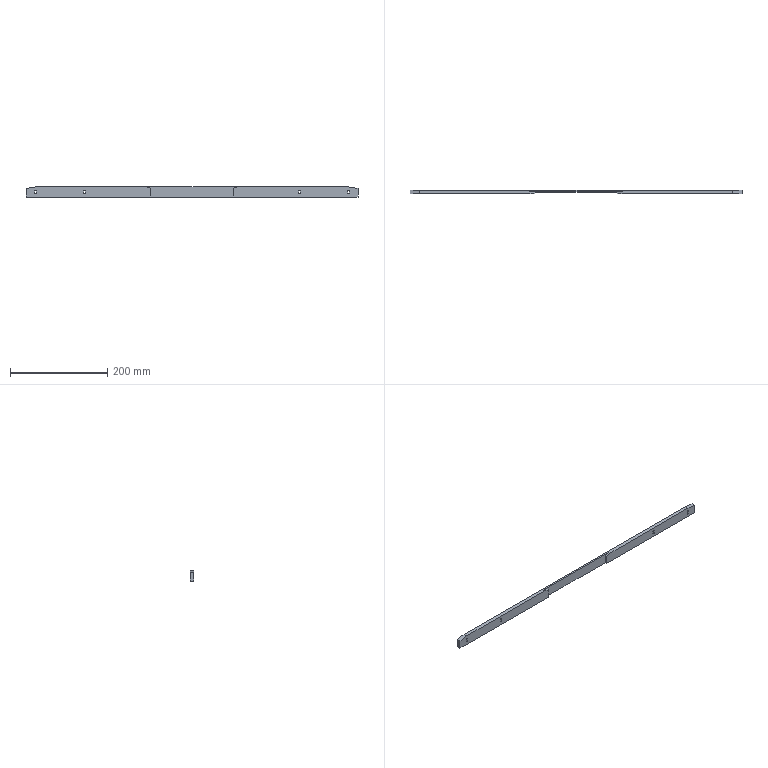Component | SolidWorks | SL010-LeftStreamline-1-1_SL010-02047858StopBarNo.3-1-2 | 1 solid | 30 faces | box 683 x 8 x 21 mm | volume 99149 mm3 | plane 22 | cylinder 8 | commonest cylinder face diameters 3.2 x8 | material White POM
build123d program:
from build123d import *

# Parameters (mm, degrees)
SKETCH1_W           = 683
SKETCH1_H           = 21
BOSS_EXTRUDE1_DEPTH = 8
CUT_EXTRUDE1_DEPTH  = 342.755
CHAMFER1_SIZE       = 3
CHAMFER1_SIZE2      = 20
CHAMFER2_SIZE       = 20
CHAMFER2_SIZE2      = 3
SKETCH4_W           = 169.5
SKETCH4_H           = 4
CUT_EXTRUDE3_DEPTH  = 343.239
CHAMFER3_SIZE       = 10
CHAMFER3_SIZE2      = 2.679


with BuildPart() as part:
    # Sketch1 → Boss-Extrude1 (new body)
    with BuildSketch(Plane.XY):
        Rectangle(SKETCH1_W, SKETCH1_H)
    extrude(amount=BOSS_EXTRUDE1_DEPTH)

    # Sketch2 → Cut-Extrude1 (cut, through all)
    with BuildSketch(Plane.XY.offset(8)):
        with BuildLine():
            Line((223.1, 2.5), (223.1, -2.5))
            ThreePointArc((223.1, -2.5), (221.5, -4.1), (219.9, -2.5))
            Line((219.9, -2.5), (219.9, 2.5))
            ThreePointArc((219.9, 2.5), (221.5, 4.1), (223.1, 2.5))
        make_face()
        with BuildLine():
            Line((323.1, 2.5), (323.1, -2.5))
            ThreePointArc((323.1, -2.5), (321.5, -4.1), (319.9, -2.5))
            Line((319.9, -2.5), (319.9, 2.5))
            ThreePointArc((319.9, 2.5), (321.5, 4.1), (323.1, 2.5))
        make_face()
        with BuildLine():
            Line((-323.1, 2.5), (-323.1, -2.5))
            ThreePointArc((-323.1, -2.5), (-321.5, -4.1), (-319.9, -2.5))
            Line((-319.9, -2.5), (-319.9, 2.5))
            ThreePointArc((-319.9, 2.5), (-321.5, 4.1), (-323.1, 2.5))
        make_face()
        with BuildLine():
            Line((-223.1, 2.5), (-223.1, -2.5))
            ThreePointArc((-223.1, -2.5), (-221.5, -4.1), (-219.9, -2.5))
            Line((-219.9, -2.5), (-219.9, 2.5))
            ThreePointArc((-219.9, 2.5), (-221.5, 4.1), (-223.1, 2.5))
        make_face()
    extrude(amount=-CUT_EXTRUDE1_DEPTH, mode=Mode.SUBTRACT)

    # Chamfer1
    chamfer1_edges = [part.edges().sort_by_distance(p)[0] for p in [
        (341.5, 10.5, 4),
    ]]
    chamfer1_side = [part.faces().sort_by_distance(p)[0] for p in [
        (341.5, 0, 4),
    ]]
    chamfer(chamfer1_edges, length=CHAMFER1_SIZE, length2=CHAMFER1_SIZE2, reference=chamfer1_side[0])

    # Chamfer2
    chamfer2_edges = [part.edges().sort_by_distance(p)[0] for p in [
        (-341.5, 10.5, 4),
    ]]
    chamfer2_side = [part.faces().sort_by_distance(p)[0] for p in [
        (-10, 10.5, 4),
    ]]
    chamfer(chamfer2_edges, length=CHAMFER2_SIZE, length2=CHAMFER2_SIZE2, reference=chamfer2_side[0])

    # Sketch4 → Cut-Extrude3 (cut, through all)
    with BuildSketch(Plane(origin=(0, 10.5, 0), x_dir=(1, 0, 0), z_dir=(0, 1, 0))):
        with Locations((0, -6)):
            Rectangle(SKETCH4_W, SKETCH4_H)
    extrude(amount=-CUT_EXTRUDE3_DEPTH, mode=Mode.SUBTRACT)

    # Chamfer3
    chamfer3_edges = [part.edges().sort_by_distance(p)[0] for p in [
        (-84.75, 10.5, 6),
        (84.75, 10.5, 6),
    ]]
    chamfer3_side = [part.faces().sort_by_distance(p)[0] for p in [
        (0, 10.5, 3.696),
    ]]
    chamfer(chamfer3_edges, length=CHAMFER3_SIZE, length2=CHAMFER3_SIZE2, reference=chamfer3_side[0])


solid = part.part

# Placed as in the assembly
solid = solid.moved(Location((633.5, -101.904, -647.535), (90, 0, 0)))
STEP:
#1=COLOUR_RGB('',0.7922,0.8196,0.9333);
#2=FILL_AREA_STYLE_COLOUR('',#1);
#3=FILL_AREA_STYLE('',(#2));
#4=SURFACE_STYLE_FILL_AREA(#3);
#5=SURFACE_SIDE_STYLE('',(#4));
#6=SURFACE_STYLE_USAGE(.BOTH.,#5);
#7=PRESENTATION_STYLE_ASSIGNMENT((#6));
#8=CARTESIAN_POINT('',(21.604,-4.327,-25.907));
#9=VERTEX_POINT('',#8);
#10=CARTESIAN_POINT('',(21.604,-4.327,-25.186));
#11=VERTEX_POINT('',#10);
#12=CARTESIAN_POINT('',(21.604,-4.327,-25.907));
#13=DIRECTION('',(-0.,-0.,1.));
#14=VECTOR('',#13,39.37);
#15=LINE('',#12,#14);
#16=EDGE_CURVE('',#9,#11,#15,.T.);
#17=ORIENTED_EDGE('',*,*,#16,.T.);
#18=CARTESIAN_POINT('',(21.211,-4.327,-25.08));
#19=VERTEX_POINT('',#18);
#20=CARTESIAN_POINT('',(24.794,-4.327,-26.04));
#21=DIRECTION('',(-0.9659,0.,0.2588));
#22=VECTOR('',#21,39.37);
#23=LINE('',#20,#22);
#24=EDGE_CURVE('',#11,#19,#23,.T.);
#25=ORIENTED_EDGE('',*,*,#24,.T.);
#26=CARTESIAN_POINT('',(12.283,-4.327,-25.08));
#27=VERTEX_POINT('',#26);
#28=CARTESIAN_POINT('',(11.496,-4.327,-25.08));
#29=DIRECTION('',(-1.,0.,-0.));
#30=VECTOR('',#29,39.37);
#31=LINE('',#28,#30);
#32=EDGE_CURVE('',#19,#27,#31,.T.);
#33=ORIENTED_EDGE('',*,*,#32,.T.);
#34=CARTESIAN_POINT('',(11.496,-4.327,-25.198));
#35=VERTEX_POINT('',#34);
#36=CARTESIAN_POINT('',(24.602,-4.327,-23.232));
#37=DIRECTION('',(-0.9889,0.,-0.1483));
#38=VECTOR('',#37,39.37);
#39=LINE('',#36,#38);
#40=EDGE_CURVE('',#27,#35,#39,.T.);
#41=ORIENTED_EDGE('',*,*,#40,.T.);
#42=CARTESIAN_POINT('',(11.496,-4.327,-25.907));
#43=VERTEX_POINT('',#42);
#44=CARTESIAN_POINT('',(11.496,-4.327,-25.08));
#45=DIRECTION('',(0.,0.,-1.));
#46=VECTOR('',#45,39.37);
#47=LINE('',#44,#46);
#48=EDGE_CURVE('',#35,#43,#47,.T.);
#49=ORIENTED_EDGE('',*,*,#48,.T.);
#50=CARTESIAN_POINT('',(11.496,-4.327,-25.907));
#51=DIRECTION('',(1.,-0.,0.));
#52=VECTOR('',#51,39.37);
#53=LINE('',#50,#52);
#54=EDGE_CURVE('',#43,#9,#53,.T.);
#55=ORIENTED_EDGE('',*,*,#54,.T.);
#56=EDGE_LOOP('',(#17,#25,#33,#41,#49,#55));
#57=FACE_OUTER_BOUND('',#56,.T.);
#58=CARTESIAN_POINT('',(12.346,-4.327,-25.395));
#59=VERTEX_POINT('',#58);
#60=CARTESIAN_POINT('',(12.22,-4.327,-25.395));
#61=VERTEX_POINT('',#60);
#62=CARTESIAN_POINT('',(12.283,-4.327,-25.395));
#63=DIRECTION('',(-0.,-1.,0.));
#64=DIRECTION('',(-1.,0.,0.));
#65=AXIS2_PLACEMENT_3D('',#62,#63,#64);
#66=CIRCLE('',#65,0.06299);
#67=EDGE_CURVE('',#59,#61,#66,.T.);
#68=ORIENTED_EDGE('',*,*,#67,.F.);
#69=CARTESIAN_POINT('',(12.346,-4.327,-25.592));
#70=VERTEX_POINT('',#69);
#71=CARTESIAN_POINT('',(12.346,-4.327,-25.395));
#72=DIRECTION('',(-0.,-0.,1.));
#73=VECTOR('',#72,39.37);
#74=LINE('',#71,#73);
#75=EDGE_CURVE('',#70,#59,#74,.T.);
#76=ORIENTED_EDGE('',*,*,#75,.F.);
#77=CARTESIAN_POINT('',(12.22,-4.327,-25.592));
#78=VERTEX_POINT('',#77);
#79=CARTESIAN_POINT('',(12.283,-4.327,-25.592));
#80=DIRECTION('',(-0.,-1.,0.));
#81=DIRECTION('',(-1.,0.,0.));
#82=AXIS2_PLACEMENT_3D('',#79,#80,#81);
#83=CIRCLE('',#82,0.06299);
#84=EDGE_CURVE('',#78,#70,#83,.T.);
#85=ORIENTED_EDGE('',*,*,#84,.F.);
#86=CARTESIAN_POINT('',(12.22,-4.327,-25.395));
#87=DIRECTION('',(0.,0.,-1.));
#88=VECTOR('',#87,39.37);
#89=LINE('',#86,#88);
#90=EDGE_CURVE('',#61,#78,#89,.T.);
#91=ORIENTED_EDGE('',*,*,#90,.F.);
#92=EDGE_LOOP('',(#68,#76,#85,#91));
#93=FACE_BOUND('',#92,.T.);
#94=CARTESIAN_POINT('',(16.283,-4.327,-25.395));
#95=VERTEX_POINT('',#94);
#96=CARTESIAN_POINT('',(16.157,-4.327,-25.395));
#97=VERTEX_POINT('',#96);
#98=CARTESIAN_POINT('',(16.22,-4.327,-25.395));
#99=DIRECTION('',(-0.,-1.,0.));
#100=DIRECTION('',(-1.,0.,0.));
#101=AXIS2_PLACEMENT_3D('',#98,#99,#100);
#102=CIRCLE('',#101,0.06299);
#103=EDGE_CURVE('',#95,#97,#102,.T.);
#104=ORIENTED_EDGE('',*,*,#103,.F.);
#105=CARTESIAN_POINT('',(16.283,-4.327,-25.592));
#106=VERTEX_POINT('',#105);
#107=CARTESIAN_POINT('',(16.283,-4.327,-25.395));
#108=DIRECTION('',(-0.,-0.,1.));
#109=VECTOR('',#108,39.37);
#110=LINE('',#107,#109);
#111=EDGE_CURVE('',#106,#95,#110,.T.);
#112=ORIENTED_EDGE('',*,*,#111,.F.);
#113=CARTESIAN_POINT('',(16.157,-4.327,-25.592));
#114=VERTEX_POINT('',#113);
#115=CARTESIAN_POINT('',(16.22,-4.327,-25.592));
#116=DIRECTION('',(-0.,-1.,0.));
#117=DIRECTION('',(-1.,0.,0.));
#118=AXIS2_PLACEMENT_3D('',#115,#116,#117);
#119=CIRCLE('',#118,0.06299);
#120=EDGE_CURVE('',#114,#106,#119,.T.);
#121=ORIENTED_EDGE('',*,*,#120,.F.);
#122=CARTESIAN_POINT('',(16.157,-4.327,-25.395));
#123=DIRECTION('',(0.,0.,-1.));
#124=VECTOR('',#123,39.37);
#125=LINE('',#122,#124);
#126=EDGE_CURVE('',#97,#114,#125,.T.);
#127=ORIENTED_EDGE('',*,*,#126,.F.);
#128=EDGE_LOOP('',(#104,#112,#121,#127));
#129=FACE_BOUND('',#128,.T.);
#130=CARTESIAN_POINT('',(24.941,-4.327,-25.494));
#131=DIRECTION('',(-0.,-1.,0.));
#132=DIRECTION('',(1.,-0.,0.));
#133=AXIS2_PLACEMENT_3D('',#130,#131,#132);
#134=PLANE('',#133);
#135=ADVANCED_FACE('',(#57,#93,#129),#134,.T.);
#136=CARTESIAN_POINT('',(38.386,-4.012,-25.907));
#137=VERTEX_POINT('',#136);
#138=CARTESIAN_POINT('',(38.386,-4.012,-25.198));
#139=VERTEX_POINT('',#138);
#140=CARTESIAN_POINT('',(38.386,-4.012,-25.08));
#141=DIRECTION('',(-0.,-0.,1.));
#142=VECTOR('',#141,39.37);
#143=LINE('',#140,#142);
#144=EDGE_CURVE('',#137,#139,#143,.T.);
#145=ORIENTED_EDGE('',*,*,#144,.T.);
#146=CARTESIAN_POINT('',(38.386,-4.327,-25.198));
#147=VERTEX_POINT('',#146);
#148=CARTESIAN_POINT('',(38.386,-4.327,-25.198));
#149=DIRECTION('',(-0.,-1.,0.));
#150=VECTOR('',#149,39.37);
#151=LINE('',#148,#150);
#152=EDGE_CURVE('',#139,#147,#151,.T.);
#153=ORIENTED_EDGE('',*,*,#152,.T.);
#154=CARTESIAN_POINT('',(38.386,-4.327,-25.907));
#155=VERTEX_POINT('',#154);
#156=CARTESIAN_POINT('',(38.386,-4.327,-25.08));
#157=DIRECTION('',(-0.,-0.,1.));
#158=VECTOR('',#157,39.37);
#159=LINE('',#156,#158);
#160=EDGE_CURVE('',#155,#147,#159,.T.);
#161=ORIENTED_EDGE('',*,*,#160,.F.);
#162=CARTESIAN_POINT('',(38.386,-4.327,-25.907));
#163=DIRECTION('',(0.,1.,-0.));
#164=VECTOR('',#163,39.37);
#165=LINE('',#162,#164);
#166=EDGE_CURVE('',#155,#137,#165,.T.);
#167=ORIENTED_EDGE('',*,*,#166,.T.);
#168=EDGE_LOOP('',(#145,#153,#161,#167));
#169=FACE_OUTER_BOUND('',#168,.T.);
#170=CARTESIAN_POINT('',(38.386,-4.327,-25.08));
#171=DIRECTION('',(-1.,0.,-0.));
#172=DIRECTION('',(-0.,-1.,0.));
#173=AXIS2_PLACEMENT_3D('',#170,#171,#172);
#174=PLANE('',#173);
#175=ADVANCED_FACE('',(#169),#174,.F.);
#176=CARTESIAN_POINT('',(28.671,-4.169,-25.08));
#177=VERTEX_POINT('',#176);
#178=CARTESIAN_POINT('',(21.211,-4.169,-25.08));
#179=VERTEX_POINT('',#178);
#180=CARTESIAN_POINT('',(21.604,-4.169,-25.08));
#181=DIRECTION('',(-1.,-0.,-0.));
#182=VECTOR('',#181,39.37);
#183=LINE('',#180,#182);
#184=EDGE_CURVE('',#177,#179,#183,.T.);
#185=ORIENTED_EDGE('',*,*,#184,.F.);
#186=CARTESIAN_POINT('',(28.671,-4.327,-25.08));
#187=VERTEX_POINT('',#186);
#188=CARTESIAN_POINT('',(28.671,-4.327,-25.08));
#189=DIRECTION('',(-0.,-1.,0.));
#190=VECTOR('',#189,39.37);
#191=LINE('',#188,#190);
#192=EDGE_CURVE('',#177,#187,#191,.T.);
#193=ORIENTED_EDGE('',*,*,#192,.T.);
#194=CARTESIAN_POINT('',(37.598,-4.327,-25.08));
#195=VERTEX_POINT('',#194);
#196=CARTESIAN_POINT('',(11.496,-4.327,-25.08));
#197=DIRECTION('',(-1.,0.,-0.));
#198=VECTOR('',#197,39.37);
#199=LINE('',#196,#198);
#200=EDGE_CURVE('',#195,#187,#199,.T.);
#201=ORIENTED_EDGE('',*,*,#200,.F.);
#202=CARTESIAN_POINT('',(37.598,-4.012,-25.08));
#203=VERTEX_POINT('',#202);
#204=CARTESIAN_POINT('',(37.598,-4.327,-25.08));
#205=DIRECTION('',(0.,1.,-0.));
#206=VECTOR('',#205,39.37);
#207=LINE('',#204,#206);
#208=EDGE_CURVE('',#195,#203,#207,.T.);
#209=ORIENTED_EDGE('',*,*,#208,.T.);
#210=CARTESIAN_POINT('',(12.283,-4.012,-25.08));
#211=VERTEX_POINT('',#210);
#212=CARTESIAN_POINT('',(11.496,-4.012,-25.08));
#213=DIRECTION('',(-1.,0.,-0.));
#214=VECTOR('',#213,39.37);
#215=LINE('',#212,#214);
#216=EDGE_CURVE('',#203,#211,#215,.T.);
#217=ORIENTED_EDGE('',*,*,#216,.T.);
#218=CARTESIAN_POINT('',(12.283,-4.327,-25.08));
#219=DIRECTION('',(-0.,-1.,0.));
#220=VECTOR('',#219,39.37);
#221=LINE('',#218,#220);
#222=EDGE_CURVE('',#211,#27,#221,.T.);
#223=ORIENTED_EDGE('',*,*,#222,.T.);
#224=ORIENTED_EDGE('',*,*,#32,.F.);
#225=CARTESIAN_POINT('',(21.211,-4.327,-25.08));
#226=DIRECTION('',(0.,1.,-0.));
#227=VECTOR('',#226,39.37);
#228=LINE('',#225,#227);
#229=EDGE_CURVE('',#19,#179,#228,.T.);
#230=ORIENTED_EDGE('',*,*,#229,.T.);
#231=EDGE_LOOP('',(#185,#193,#201,#209,#217,#223,#224,#230));
#232=FACE_OUTER_BOUND('',#231,.T.);
#233=CARTESIAN_POINT('',(11.496,-4.327,-25.08));
#234=DIRECTION('',(0.,-0.,-1.));
#235=DIRECTION('',(0.,1.,-0.));
#236=AXIS2_PLACEMENT_3D('',#233,#234,#235);
#237=PLANE('',#236);
#238=ADVANCED_FACE('',(#232),#237,.F.);
#239=ORIENTED_EDGE('',*,*,#48,.F.);
#240=CARTESIAN_POINT('',(11.496,-4.012,-25.198));
#241=VERTEX_POINT('',#240);
#242=CARTESIAN_POINT('',(11.496,-4.327,-25.198));
#243=DIRECTION('',(0.,1.,-0.));
#244=VECTOR('',#243,39.37);
#245=LINE('',#242,#244);
#246=EDGE_CURVE('',#35,#241,#245,.T.);
#247=ORIENTED_EDGE('',*,*,#246,.T.);
#248=CARTESIAN_POINT('',(11.496,-4.012,-25.907));
#249=VERTEX_POINT('',#248);
#250=CARTESIAN_POINT('',(11.496,-4.012,-25.08));
#251=DIRECTION('',(0.,0.,-1.));
#252=VECTOR('',#251,39.37);
#253=LINE('',#250,#252);
#254=EDGE_CURVE('',#241,#249,#253,.T.);
#255=ORIENTED_EDGE('',*,*,#254,.T.);
#256=CARTESIAN_POINT('',(11.496,-4.327,-25.907));
#257=DIRECTION('',(0.,1.,-0.));
#258=VECTOR('',#257,39.37);
#259=LINE('',#256,#258);
#260=EDGE_CURVE('',#43,#249,#259,.T.);
#261=ORIENTED_EDGE('',*,*,#260,.F.);
#262=EDGE_LOOP('',(#239,#247,#255,#261));
#263=FACE_OUTER_BOUND('',#262,.T.);
#264=CARTESIAN_POINT('',(11.496,-4.327,-25.08));
#265=DIRECTION('',(1.,-0.,0.));
#266=DIRECTION('',(0.,1.,-0.));
#267=AXIS2_PLACEMENT_3D('',#264,#265,#266);
#268=PLANE('',#267);
#269=ADVANCED_FACE('',(#263),#268,.F.);
#270=CARTESIAN_POINT('',(28.278,-4.169,-25.907));
#271=VERTEX_POINT('',#270);
#272=CARTESIAN_POINT('',(21.604,-4.169,-25.907));
#273=VERTEX_POINT('',#272);
#274=CARTESIAN_POINT('',(21.604,-4.169,-25.907));
#275=DIRECTION('',(-1.,-0.,-0.));
#276=VECTOR('',#275,39.37);
#277=LINE('',#274,#276);
#278=EDGE_CURVE('',#271,#273,#277,.T.);
#279=ORIENTED_EDGE('',*,*,#278,.T.);
#280=CARTESIAN_POINT('',(21.604,-4.327,-25.907));
#281=DIRECTION('',(-0.,-1.,0.));
#282=VECTOR('',#281,39.37);
#283=LINE('',#280,#282);
#284=EDGE_CURVE('',#273,#9,#283,.T.);
#285=ORIENTED_EDGE('',*,*,#284,.T.);
#286=ORIENTED_EDGE('',*,*,#54,.F.);
#287=ORIENTED_EDGE('',*,*,#260,.T.);
#288=CARTESIAN_POINT('',(11.496,-4.012,-25.907));
#289=DIRECTION('',(1.,-0.,0.));
#290=VECTOR('',#289,39.37);
#291=LINE('',#288,#290);
#292=EDGE_CURVE('',#249,#137,#291,.T.);
#293=ORIENTED_EDGE('',*,*,#292,.T.);
#294=ORIENTED_EDGE('',*,*,#166,.F.);
#295=CARTESIAN_POINT('',(28.278,-4.327,-25.907));
#296=VERTEX_POINT('',#295);
#297=CARTESIAN_POINT('',(11.496,-4.327,-25.907));
#298=DIRECTION('',(1.,-0.,0.));
#299=VECTOR('',#298,39.37);
#300=LINE('',#297,#299);
#301=EDGE_CURVE('',#296,#155,#300,.T.);
#302=ORIENTED_EDGE('',*,*,#301,.F.);
#303=CARTESIAN_POINT('',(28.278,-4.327,-25.907));
#304=DIRECTION('',(0.,1.,-0.));
#305=VECTOR('',#304,39.37);
#306=LINE('',#303,#305);
#307=EDGE_CURVE('',#296,#271,#306,.T.);
#308=ORIENTED_EDGE('',*,*,#307,.T.);
#309=EDGE_LOOP('',(#279,#285,#286,#287,#293,#294,#302,#308));
#310=FACE_OUTER_BOUND('',#309,.T.);
#311=CARTESIAN_POINT('',(11.496,-4.327,-25.907));
#312=DIRECTION('',(-0.,0.,1.));
#313=DIRECTION('',(-0.,-1.,0.));
#314=AXIS2_PLACEMENT_3D('',#311,#312,#313);
#315=PLANE('',#314);
#316=ADVANCED_FACE('',(#310),#315,.F.);
#317=ORIENTED_EDGE('',*,*,#200,.T.);
#318=CARTESIAN_POINT('',(28.278,-4.327,-25.186));
#319=VERTEX_POINT('',#318);
#320=CARTESIAN_POINT('',(25.087,-4.327,-26.04));
#321=DIRECTION('',(-0.9659,0.,-0.2588));
#322=VECTOR('',#321,39.37);
#323=LINE('',#320,#322);
#324=EDGE_CURVE('',#187,#319,#323,.T.);
#325=ORIENTED_EDGE('',*,*,#324,.T.);
#326=CARTESIAN_POINT('',(28.278,-4.327,-25.907));
#327=DIRECTION('',(-0.,-0.,1.));
#328=VECTOR('',#327,39.37);
#329=LINE('',#326,#328);
#330=EDGE_CURVE('',#296,#319,#329,.T.);
#331=ORIENTED_EDGE('',*,*,#330,.F.);
#332=ORIENTED_EDGE('',*,*,#301,.T.);
#333=ORIENTED_EDGE('',*,*,#160,.T.);
#334=CARTESIAN_POINT('',(25.28,-4.327,-23.232));
#335=DIRECTION('',(-0.9889,0.,0.1483));
#336=VECTOR('',#335,39.37);
#337=LINE('',#334,#336);
#338=EDGE_CURVE('',#147,#195,#337,.T.);
#339=ORIENTED_EDGE('',*,*,#338,.T.);
#340=EDGE_LOOP('',(#317,#325,#331,#332,#333,#339));
#341=FACE_OUTER_BOUND('',#340,.T.);
#342=CARTESIAN_POINT('',(37.661,-4.327,-25.395));
#343=VERTEX_POINT('',#342);
#344=CARTESIAN_POINT('',(37.535,-4.327,-25.395));
#345=VERTEX_POINT('',#344);
#346=CARTESIAN_POINT('',(37.598,-4.327,-25.395));
#347=DIRECTION('',(-0.,-1.,0.));
#348=DIRECTION('',(1.,0.,0.));
#349=AXIS2_PLACEMENT_3D('',#346,#347,#348);
#350=CIRCLE('',#349,0.06299);
#351=EDGE_CURVE('',#343,#345,#350,.T.);
#352=ORIENTED_EDGE('',*,*,#351,.F.);
#353=CARTESIAN_POINT('',(37.661,-4.327,-25.592));
#354=VERTEX_POINT('',#353);
#355=CARTESIAN_POINT('',(37.661,-4.327,-25.395));
#356=DIRECTION('',(-0.,-0.,1.));
#357=VECTOR('',#356,39.37);
#358=LINE('',#355,#357);
#359=EDGE_CURVE('',#354,#343,#358,.T.);
#360=ORIENTED_EDGE('',*,*,#359,.F.);
#361=CARTESIAN_POINT('',(37.535,-4.327,-25.592));
#362=VERTEX_POINT('',#361);
#363=CARTESIAN_POINT('',(37.598,-4.327,-25.592));
#364=DIRECTION('',(-0.,-1.,0.));
#365=DIRECTION('',(1.,0.,0.));
#366=AXIS2_PLACEMENT_3D('',#363,#364,#365);
#367=CIRCLE('',#366,0.06299);
#368=EDGE_CURVE('',#362,#354,#367,.T.);
#369=ORIENTED_EDGE('',*,*,#368,.F.);
#370=CARTESIAN_POINT('',(37.535,-4.327,-25.395));
#371=DIRECTION('',(0.,0.,-1.));
#372=VECTOR('',#371,39.37);
#373=LINE('',#370,#372);
#374=EDGE_CURVE('',#345,#362,#373,.T.);
#375=ORIENTED_EDGE('',*,*,#374,.F.);
#376=EDGE_LOOP('',(#352,#360,#369,#375));
#377=FACE_BOUND('',#376,.T.);
#378=CARTESIAN_POINT('',(33.724,-4.327,-25.395));
#379=VERTEX_POINT('',#378);
#380=CARTESIAN_POINT('',(33.598,-4.327,-25.395));
#381=VERTEX_POINT('',#380);
#382=CARTESIAN_POINT('',(33.661,-4.327,-25.395));
#383=DIRECTION('',(-0.,-1.,0.));
#384=DIRECTION('',(1.,0.,0.));
#385=AXIS2_PLACEMENT_3D('',#382,#383,#384);
#386=CIRCLE('',#385,0.06299);
#387=EDGE_CURVE('',#379,#381,#386,.T.);
#388=ORIENTED_EDGE('',*,*,#387,.F.);
#389=CARTESIAN_POINT('',(33.724,-4.327,-25.592));
#390=VERTEX_POINT('',#389);
#391=CARTESIAN_POINT('',(33.724,-4.327,-25.395));
#392=DIRECTION('',(-0.,-0.,1.));
#393=VECTOR('',#392,39.37);
#394=LINE('',#391,#393);
#395=EDGE_CURVE('',#390,#379,#394,.T.);
#396=ORIENTED_EDGE('',*,*,#395,.F.);
#397=CARTESIAN_POINT('',(33.598,-4.327,-25.592));
#398=VERTEX_POINT('',#397);
#399=CARTESIAN_POINT('',(33.661,-4.327,-25.592));
#400=DIRECTION('',(-0.,-1.,0.));
#401=DIRECTION('',(1.,0.,0.));
#402=AXIS2_PLACEMENT_3D('',#399,#400,#401);
#403=CIRCLE('',#402,0.06299);
#404=EDGE_CURVE('',#398,#390,#403,.T.);
#405=ORIENTED_EDGE('',*,*,#404,.F.);
#406=CARTESIAN_POINT('',(33.598,-4.327,-25.395));
#407=DIRECTION('',(0.,0.,-1.));
#408=VECTOR('',#407,39.37);
#409=LINE('',#406,#408);
#410=EDGE_CURVE('',#381,#398,#409,.T.);
#411=ORIENTED_EDGE('',*,*,#410,.F.);
#412=EDGE_LOOP('',(#388,#396,#405,#411));
#413=FACE_BOUND('',#412,.T.);
#414=CARTESIAN_POINT('',(24.941,-4.327,-25.494));
#415=DIRECTION('',(-0.,-1.,0.));
#416=DIRECTION('',(1.,-0.,0.));
#417=AXIS2_PLACEMENT_3D('',#414,#415,#416);
#418=PLANE('',#417);
#419=ADVANCED_FACE('',(#341,#377,#413),#418,.T.);
#420=CARTESIAN_POINT('',(16.283,-4.012,-25.592));
#421=VERTEX_POINT('',#420);
#422=CARTESIAN_POINT('',(16.283,-4.012,-25.395));
#423=VERTEX_POINT('',#422);
#424=CARTESIAN_POINT('',(16.283,-4.012,-25.395));
#425=DIRECTION('',(-0.,-0.,1.));
#426=VECTOR('',#425,39.37);
#427=LINE('',#424,#426);
#428=EDGE_CURVE('',#421,#423,#427,.T.);
#429=ORIENTED_EDGE('',*,*,#428,.T.);
#430=CARTESIAN_POINT('',(16.157,-4.012,-25.395));
#431=VERTEX_POINT('',#430);
#432=CARTESIAN_POINT('',(16.22,-4.012,-25.395));
#433=DIRECTION('',(-0.,-1.,0.));
#434=DIRECTION('',(-1.,0.,0.));
#435=AXIS2_PLACEMENT_3D('',#432,#433,#434);
#436=CIRCLE('',#435,0.06299);
#437=EDGE_CURVE('',#423,#431,#436,.T.);
#438=ORIENTED_EDGE('',*,*,#437,.T.);
#439=CARTESIAN_POINT('',(16.157,-4.012,-25.592));
#440=VERTEX_POINT('',#439);
#441=CARTESIAN_POINT('',(16.157,-4.012,-25.395));
#442=DIRECTION('',(0.,0.,-1.));
#443=VECTOR('',#442,39.37);
#444=LINE('',#441,#443);
#445=EDGE_CURVE('',#431,#440,#444,.T.);
#446=ORIENTED_EDGE('',*,*,#445,.T.);
#447=CARTESIAN_POINT('',(16.22,-4.012,-25.592));
#448=DIRECTION('',(-0.,-1.,0.));
#449=DIRECTION('',(-1.,0.,0.));
#450=AXIS2_PLACEMENT_3D('',#447,#448,#449);
#451=CIRCLE('',#450,0.06299);
#452=EDGE_CURVE('',#440,#421,#451,.T.);
#453=ORIENTED_EDGE('',*,*,#452,.T.);
#454=EDGE_LOOP('',(#429,#438,#446,#453));
#455=FACE_BOUND('',#454,.T.);
#456=CARTESIAN_POINT('',(12.346,-4.012,-25.592));
#457=VERTEX_POINT('',#456);
#458=CARTESIAN_POINT('',(12.346,-4.012,-25.395));
#459=VERTEX_POINT('',#458);
#460=CARTESIAN_POINT('',(12.346,-4.012,-25.395));
#461=DIRECTION('',(-0.,-0.,1.));
#462=VECTOR('',#461,39.37);
#463=LINE('',#460,#462);
#464=EDGE_CURVE('',#457,#459,#463,.T.);
#465=ORIENTED_EDGE('',*,*,#464,.T.);
#466=CARTESIAN_POINT('',(12.22,-4.012,-25.395));
#467=VERTEX_POINT('',#466);
#468=CARTESIAN_POINT('',(12.283,-4.012,-25.395));
#469=DIRECTION('',(-0.,-1.,0.));
#470=DIRECTION('',(-1.,0.,0.));
#471=AXIS2_PLACEMENT_3D('',#468,#469,#470);
#472=CIRCLE('',#471,0.06299);
#473=EDGE_CURVE('',#459,#467,#472,.T.);
#474=ORIENTED_EDGE('',*,*,#473,.T.);
#475=CARTESIAN_POINT('',(12.22,-4.012,-25.592));
#476=VERTEX_POINT('',#475);
#477=CARTESIAN_POINT('',(12.22,-4.012,-25.395));
#478=DIRECTION('',(0.,0.,-1.));
#479=VECTOR('',#478,39.37);
#480=LINE('',#477,#479);
#481=EDGE_CURVE('',#467,#476,#480,.T.);
#482=ORIENTED_EDGE('',*,*,#481,.T.);
#483=CARTESIAN_POINT('',(12.283,-4.012,-25.592));
#484=DIRECTION('',(-0.,-1.,0.));
#485=DIRECTION('',(-1.,0.,0.));
#486=AXIS2_PLACEMENT_3D('',#483,#484,#485);
#487=CIRCLE('',#486,0.06299);
#488=EDGE_CURVE('',#476,#457,#487,.T.);
#489=ORIENTED_EDGE('',*,*,#488,.T.);
#490=EDGE_LOOP('',(#465,#474,#482,#489));
#491=FACE_BOUND('',#490,.T.);
#492=CARTESIAN_POINT('',(37.661,-4.012,-25.592));
#493=VERTEX_POINT('',#492);
#494=CARTESIAN_POINT('',(37.661,-4.012,-25.395));
#495=VERTEX_POINT('',#494);
#496=CARTESIAN_POINT('',(37.661,-4.012,-25.395));
#497=DIRECTION('',(-0.,-0.,1.));
#498=VECTOR('',#497,39.37);
#499=LINE('',#496,#498);
#500=EDGE_CURVE('',#493,#495,#499,.T.);
#501=ORIENTED_EDGE('',*,*,#500,.T.);
#502=CARTESIAN_POINT('',(37.535,-4.012,-25.395));
#503=VERTEX_POINT('',#502);
#504=CARTESIAN_POINT('',(37.598,-4.012,-25.395));
#505=DIRECTION('',(-0.,-1.,0.));
#506=DIRECTION('',(1.,0.,0.));
#507=AXIS2_PLACEMENT_3D('',#504,#505,#506);
#508=CIRCLE('',#507,0.06299);
#509=EDGE_CURVE('',#495,#503,#508,.T.);
#510=ORIENTED_EDGE('',*,*,#509,.T.);
#511=CARTESIAN_POINT('',(37.535,-4.012,-25.592));
#512=VERTEX_POINT('',#511);
#513=CARTESIAN_POINT('',(37.535,-4.012,-25.395));
#514=DIRECTION('',(0.,0.,-1.));
#515=VECTOR('',#514,39.37);
#516=LINE('',#513,#515);
#517=EDGE_CURVE('',#503,#512,#516,.T.);
#518=ORIENTED_EDGE('',*,*,#517,.T.);
#519=CARTESIAN_POINT('',(37.598,-4.012,-25.592));
#520=DIRECTION('',(-0.,-1.,0.));
#521=DIRECTION('',(1.,0.,0.));
#522=AXIS2_PLACEMENT_3D('',#519,#520,#521);
#523=CIRCLE('',#522,0.06299);
#524=EDGE_CURVE('',#512,#493,#523,.T.);
#525=ORIENTED_EDGE('',*,*,#524,.T.);
#526=EDGE_LOOP('',(#501,#510,#518,#525));
#527=FACE_BOUND('',#526,.T.);
#528=CARTESIAN_POINT('',(33.724,-4.012,-25.592));
#529=VERTEX_POINT('',#528);
#530=CARTESIAN_POINT('',(33.724,-4.012,-25.395));
#531=VERTEX_POINT('',#530);
#532=CARTESIAN_POINT('',(33.724,-4.012,-25.395));
#533=DIRECTION('',(-0.,-0.,1.));
#534=VECTOR('',#533,39.37);
#535=LINE('',#532,#534);
#536=EDGE_CURVE('',#529,#531,#535,.T.);
#537=ORIENTED_EDGE('',*,*,#536,.T.);
#538=CARTESIAN_POINT('',(33.598,-4.012,-25.395));
#539=VERTEX_POINT('',#538);
#540=CARTESIAN_POINT('',(33.661,-4.012,-25.395));
#541=DIRECTION('',(-0.,-1.,0.));
#542=DIRECTION('',(1.,0.,0.));
#543=AXIS2_PLACEMENT_3D('',#540,#541,#542);
#544=CIRCLE('',#543,0.06299);
#545=EDGE_CURVE('',#531,#539,#544,.T.);
#546=ORIENTED_EDGE('',*,*,#545,.T.);
#547=CARTESIAN_POINT('',(33.598,-4.012,-25.592));
#548=VERTEX_POINT('',#547);
#549=CARTESIAN_POINT('',(33.598,-4.012,-25.395));
#550=DIRECTION('',(0.,0.,-1.));
#551=VECTOR('',#550,39.37);
#552=LINE('',#549,#551);
#553=EDGE_CURVE('',#539,#548,#552,.T.);
#554=ORIENTED_EDGE('',*,*,#553,.T.);
#555=CARTESIAN_POINT('',(33.661,-4.012,-25.592));
#556=DIRECTION('',(-0.,-1.,0.));
#557=DIRECTION('',(1.,0.,0.));
#558=AXIS2_PLACEMENT_3D('',#555,#556,#557);
#559=CIRCLE('',#558,0.06299);
#560=EDGE_CURVE('',#548,#529,#559,.T.);
#561=ORIENTED_EDGE('',*,*,#560,.T.);
#562=EDGE_LOOP('',(#537,#546,#554,#561));
#563=FACE_BOUND('',#562,.T.);
#564=ORIENTED_EDGE('',*,*,#254,.F.);
#565=CARTESIAN_POINT('',(11.496,-4.012,-25.198));
#566=DIRECTION('',(0.9889,-0.,0.1483));
#567=VECTOR('',#566,39.37);
#568=LINE('',#565,#567);
#569=EDGE_CURVE('',#241,#211,#568,.T.);
#570=ORIENTED_EDGE('',*,*,#569,.T.);
#571=ORIENTED_EDGE('',*,*,#216,.F.);
#572=CARTESIAN_POINT('',(37.598,-4.012,-25.08));
#573=DIRECTION('',(0.9889,-0.,-0.1483));
#574=VECTOR('',#573,39.37);
#575=LINE('',#572,#574);
#576=EDGE_CURVE('',#203,#139,#575,.T.);
#577=ORIENTED_EDGE('',*,*,#576,.T.);
#578=ORIENTED_EDGE('',*,*,#144,.F.);
#579=ORIENTED_EDGE('',*,*,#292,.F.);
#580=EDGE_LOOP('',(#564,#570,#571,#577,#578,#579));
#581=FACE_OUTER_BOUND('',#580,.T.);
#582=CARTESIAN_POINT('',(24.941,-4.012,-25.494));
#583=DIRECTION('',(-0.,-1.,0.));
#584=DIRECTION('',(1.,-0.,0.));
#585=AXIS2_PLACEMENT_3D('',#582,#583,#584);
#586=PLANE('',#585);
#587=ADVANCED_FACE('',(#455,#491,#527,#563,#581),#586,.F.);
#588=ORIENTED_EDGE('',*,*,#387,.T.);
#589=CARTESIAN_POINT('',(33.598,-4.012,-25.395));
#590=DIRECTION('',(-0.,-1.,0.));
#591=VECTOR('',#590,39.37);
#592=LINE('',#589,#591);
#593=EDGE_CURVE('',#539,#381,#592,.T.);
#594=ORIENTED_EDGE('',*,*,#593,.F.);
#595=ORIENTED_EDGE('',*,*,#545,.F.);
#596=CARTESIAN_POINT('',(33.724,-4.012,-25.395));
#597=DIRECTION('',(-0.,-1.,0.));
#598=VECTOR('',#597,39.37);
#599=LINE('',#596,#598);
#600=EDGE_CURVE('',#531,#379,#599,.T.);
#601=ORIENTED_EDGE('',*,*,#600,.T.);
#602=EDGE_LOOP('',(#588,#594,#595,#601));
#603=FACE_OUTER_BOUND('',#602,.T.);
#604=CARTESIAN_POINT('',(33.661,-4.012,-25.395));
#605=DIRECTION('',(-0.,-1.,0.));
#606=DIRECTION('',(1.,0.,0.));
#607=AXIS2_PLACEMENT_3D('',#604,#605,#606);
#608=CYLINDRICAL_SURFACE('',#607,0.06299);
#609=ADVANCED_FACE('',(#603),#608,.F.);
#610=ORIENTED_EDGE('',*,*,#395,.T.);
#611=ORIENTED_EDGE('',*,*,#600,.F.);
#612=ORIENTED_EDGE('',*,*,#536,.F.);
#613=CARTESIAN_POINT('',(33.724,-4.012,-25.592));
#614=DIRECTION('',(-0.,-1.,0.));
#615=VECTOR('',#614,39.37);
#616=LINE('',#613,#615);
#617=EDGE_CURVE('',#529,#390,#616,.T.);
#618=ORIENTED_EDGE('',*,*,#617,.T.);
#619=EDGE_LOOP('',(#610,#611,#612,#618));
#620=FACE_OUTER_BOUND('',#619,.T.);
#621=CARTESIAN_POINT('',(33.724,-4.012,-25.395));
#622=DIRECTION('',(1.,-0.,0.));
#623=DIRECTION('',(0.,1.,-0.));
#624=AXIS2_PLACEMENT_3D('',#621,#622,#623);
#625=PLANE('',#624);
#626=ADVANCED_FACE('',(#620),#625,.F.);
#627=ORIENTED_EDGE('',*,*,#404,.T.);
#628=ORIENTED_EDGE('',*,*,#617,.F.);
#629=ORIENTED_EDGE('',*,*,#560,.F.);
#630=CARTESIAN_POINT('',(33.598,-4.012,-25.592));
#631=DIRECTION('',(-0.,-1.,0.));
#632=VECTOR('',#631,39.37);
#633=LINE('',#630,#632);
#634=EDGE_CURVE('',#548,#398,#633,.T.);
#635=ORIENTED_EDGE('',*,*,#634,.T.);
#636=EDGE_LOOP('',(#627,#628,#629,#635));
#637=FACE_OUTER_BOUND('',#636,.T.);
#638=CARTESIAN_POINT('',(33.661,-4.012,-25.592));
#639=DIRECTION('',(-0.,-1.,0.));
#640=DIRECTION('',(1.,0.,0.));
#641=AXIS2_PLACEMENT_3D('',#638,#639,#640);
#642=CYLINDRICAL_SURFACE('',#641,0.06299);
#643=ADVANCED_FACE('',(#637),#642,.F.);
#644=ORIENTED_EDGE('',*,*,#410,.T.);
#645=ORIENTED_EDGE('',*,*,#634,.F.);
#646=ORIENTED_EDGE('',*,*,#553,.F.);
#647=ORIENTED_EDGE('',*,*,#593,.T.);
#648=EDGE_LOOP('',(#644,#645,#646,#647));
#649=FACE_OUTER_BOUND('',#648,.T.);
#650=CARTESIAN_POINT('',(33.598,-4.012,-25.395));
#651=DIRECTION('',(-1.,0.,-0.));
#652=DIRECTION('',(-0.,-1.,0.));
#653=AXIS2_PLACEMENT_3D('',#650,#651,#652);
#654=PLANE('',#653);
#655=ADVANCED_FACE('',(#649),#654,.F.);
#656=ORIENTED_EDGE('',*,*,#351,.T.);
#657=CARTESIAN_POINT('',(37.535,-4.012,-25.395));
#658=DIRECTION('',(-0.,-1.,0.));
#659=VECTOR('',#658,39.37);
#660=LINE('',#657,#659);
#661=EDGE_CURVE('',#503,#345,#660,.T.);
#662=ORIENTED_EDGE('',*,*,#661,.F.);
#663=ORIENTED_EDGE('',*,*,#509,.F.);
#664=CARTESIAN_POINT('',(37.661,-4.012,-25.395));
#665=DIRECTION('',(-0.,-1.,0.));
#666=VECTOR('',#665,39.37);
#667=LINE('',#664,#666);
#668=EDGE_CURVE('',#495,#343,#667,.T.);
#669=ORIENTED_EDGE('',*,*,#668,.T.);
#670=EDGE_LOOP('',(#656,#662,#663,#669));
#671=FACE_OUTER_BOUND('',#670,.T.);
#672=CARTESIAN_POINT('',(37.598,-4.012,-25.395));
#673=DIRECTION('',(-0.,-1.,0.));
#674=DIRECTION('',(1.,0.,0.));
#675=AXIS2_PLACEMENT_3D('',#672,#673,#674);
#676=CYLINDRICAL_SURFACE('',#675,0.06299);
#677=ADVANCED_FACE('',(#671),#676,.F.);
#678=ORIENTED_EDGE('',*,*,#359,.T.);
#679=ORIENTED_EDGE('',*,*,#668,.F.);
#680=ORIENTED_EDGE('',*,*,#500,.F.);
#681=CARTESIAN_POINT('',(37.661,-4.012,-25.592));
#682=DIRECTION('',(-0.,-1.,0.));
#683=VECTOR('',#682,39.37);
#684=LINE('',#681,#683);
#685=EDGE_CURVE('',#493,#354,#684,.T.);
#686=ORIENTED_EDGE('',*,*,#685,.T.);
#687=EDGE_LOOP('',(#678,#679,#680,#686));
#688=FACE_OUTER_BOUND('',#687,.T.);
#689=CARTESIAN_POINT('',(37.661,-4.012,-25.395));
#690=DIRECTION('',(1.,-0.,0.));
#691=DIRECTION('',(0.,1.,-0.));
#692=AXIS2_PLACEMENT_3D('',#689,#690,#691);
#693=PLANE('',#692);
#694=ADVANCED_FACE('',(#688),#693,.F.);
#695=ORIENTED_EDGE('',*,*,#368,.T.);
#696=ORIENTED_EDGE('',*,*,#685,.F.);
#697=ORIENTED_EDGE('',*,*,#524,.F.);
#698=CARTESIAN_POINT('',(37.535,-4.012,-25.592));
#699=DIRECTION('',(-0.,-1.,0.));
#700=VECTOR('',#699,39.37);
#701=LINE('',#698,#700);
#702=EDGE_CURVE('',#512,#362,#701,.T.);
#703=ORIENTED_EDGE('',*,*,#702,.T.);
#704=EDGE_LOOP('',(#695,#696,#697,#703));
#705=FACE_OUTER_BOUND('',#704,.T.);
#706=CARTESIAN_POINT('',(37.598,-4.012,-25.592));
#707=DIRECTION('',(-0.,-1.,0.));
#708=DIRECTION('',(1.,0.,0.));
#709=AXIS2_PLACEMENT_3D('',#706,#707,#708);
#710=CYLINDRICAL_SURFACE('',#709,0.06299);
#711=ADVANCED_FACE('',(#705),#710,.F.);
#712=ORIENTED_EDGE('',*,*,#374,.T.);
#713=ORIENTED_EDGE('',*,*,#702,.F.);
#714=ORIENTED_EDGE('',*,*,#517,.F.);
#715=ORIENTED_EDGE('',*,*,#661,.T.);
#716=EDGE_LOOP('',(#712,#713,#714,#715));
#717=FACE_OUTER_BOUND('',#716,.T.);
#718=CARTESIAN_POINT('',(37.535,-4.012,-25.395));
#719=DIRECTION('',(-1.,0.,-0.));
#720=DIRECTION('',(-0.,-1.,0.));
#721=AXIS2_PLACEMENT_3D('',#718,#719,#720);
#722=PLANE('',#721);
#723=ADVANCED_FACE('',(#717),#722,.F.);
#724=ORIENTED_EDGE('',*,*,#67,.T.);
#725=CARTESIAN_POINT('',(12.22,-4.012,-25.395));
#726=DIRECTION('',(-0.,-1.,0.));
#727=VECTOR('',#726,39.37);
#728=LINE('',#725,#727);
#729=EDGE_CURVE('',#467,#61,#728,.T.);
#730=ORIENTED_EDGE('',*,*,#729,.F.);
#731=ORIENTED_EDGE('',*,*,#473,.F.);
#732=CARTESIAN_POINT('',(12.346,-4.012,-25.395));
#733=DIRECTION('',(-0.,-1.,0.));
#734=VECTOR('',#733,39.37);
#735=LINE('',#732,#734);
#736=EDGE_CURVE('',#459,#59,#735,.T.);
#737=ORIENTED_EDGE('',*,*,#736,.T.);
#738=EDGE_LOOP('',(#724,#730,#731,#737));
#739=FACE_OUTER_BOUND('',#738,.T.);
#740=CARTESIAN_POINT('',(12.283,-4.012,-25.395));
#741=DIRECTION('',(-0.,-1.,0.));
#742=DIRECTION('',(1.,0.,0.));
#743=AXIS2_PLACEMENT_3D('',#740,#741,#742);
#744=CYLINDRICAL_SURFACE('',#743,0.06299);
#745=ADVANCED_FACE('',(#739),#744,.F.);
#746=ORIENTED_EDGE('',*,*,#75,.T.);
#747=ORIENTED_EDGE('',*,*,#736,.F.);
#748=ORIENTED_EDGE('',*,*,#464,.F.);
#749=CARTESIAN_POINT('',(12.346,-4.012,-25.592));
#750=DIRECTION('',(-0.,-1.,0.));
#751=VECTOR('',#750,39.37);
#752=LINE('',#749,#751);
#753=EDGE_CURVE('',#457,#70,#752,.T.);
#754=ORIENTED_EDGE('',*,*,#753,.T.);
#755=EDGE_LOOP('',(#746,#747,#748,#754));
#756=FACE_OUTER_BOUND('',#755,.T.);
#757=CARTESIAN_POINT('',(12.346,-4.012,-25.395));
#758=DIRECTION('',(1.,-0.,0.));
#759=DIRECTION('',(0.,1.,-0.));
#760=AXIS2_PLACEMENT_3D('',#757,#758,#759);
#761=PLANE('',#760);
#762=ADVANCED_FACE('',(#756),#761,.F.);
#763=ORIENTED_EDGE('',*,*,#84,.T.);
#764=ORIENTED_EDGE('',*,*,#753,.F.);
#765=ORIENTED_EDGE('',*,*,#488,.F.);
#766=CARTESIAN_POINT('',(12.22,-4.012,-25.592));
#767=DIRECTION('',(-0.,-1.,0.));
#768=VECTOR('',#767,39.37);
#769=LINE('',#766,#768);
#770=EDGE_CURVE('',#476,#78,#769,.T.);
#771=ORIENTED_EDGE('',*,*,#770,.T.);
#772=EDGE_LOOP('',(#763,#764,#765,#771));
#773=FACE_OUTER_BOUND('',#772,.T.);
#774=CARTESIAN_POINT('',(12.283,-4.012,-25.592));
#775=DIRECTION('',(-0.,-1.,0.));
#776=DIRECTION('',(1.,0.,0.));
#777=AXIS2_PLACEMENT_3D('',#774,#775,#776);
#778=CYLINDRICAL_SURFACE('',#777,0.06299);
#779=ADVANCED_FACE('',(#773),#778,.F.);
#780=ORIENTED_EDGE('',*,*,#90,.T.);
#781=ORIENTED_EDGE('',*,*,#770,.F.);
#782=ORIENTED_EDGE('',*,*,#481,.F.);
#783=ORIENTED_EDGE('',*,*,#729,.T.);
#784=EDGE_LOOP('',(#780,#781,#782,#783));
#785=FACE_OUTER_BOUND('',#784,.T.);
#786=CARTESIAN_POINT('',(12.22,-4.012,-25.395));
#787=DIRECTION('',(-1.,0.,-0.));
#788=DIRECTION('',(-0.,-1.,0.));
#789=AXIS2_PLACEMENT_3D('',#786,#787,#788);
#790=PLANE('',#789);
#791=ADVANCED_FACE('',(#785),#790,.F.);
#792=ORIENTED_EDGE('',*,*,#103,.T.);
#793=CARTESIAN_POINT('',(16.157,-4.012,-25.395));
#794=DIRECTION('',(-0.,-1.,0.));
#795=VECTOR('',#794,39.37);
#796=LINE('',#793,#795);
#797=EDGE_CURVE('',#431,#97,#796,.T.);
#798=ORIENTED_EDGE('',*,*,#797,.F.);
#799=ORIENTED_EDGE('',*,*,#437,.F.);
#800=CARTESIAN_POINT('',(16.283,-4.012,-25.395));
#801=DIRECTION('',(-0.,-1.,0.));
#802=VECTOR('',#801,39.37);
#803=LINE('',#800,#802);
#804=EDGE_CURVE('',#423,#95,#803,.T.);
#805=ORIENTED_EDGE('',*,*,#804,.T.);
#806=EDGE_LOOP('',(#792,#798,#799,#805));
#807=FACE_OUTER_BOUND('',#806,.T.);
#808=CARTESIAN_POINT('',(16.22,-4.012,-25.395));
#809=DIRECTION('',(-0.,-1.,0.));
#810=DIRECTION('',(1.,0.,0.));
#811=AXIS2_PLACEMENT_3D('',#808,#809,#810);
#812=CYLINDRICAL_SURFACE('',#811,0.06299);
#813=ADVANCED_FACE('',(#807),#812,.F.);
#814=ORIENTED_EDGE('',*,*,#111,.T.);
#815=ORIENTED_EDGE('',*,*,#804,.F.);
#816=ORIENTED_EDGE('',*,*,#428,.F.);
#817=CARTESIAN_POINT('',(16.283,-4.012,-25.592));
#818=DIRECTION('',(-0.,-1.,0.));
#819=VECTOR('',#818,39.37);
#820=LINE('',#817,#819);
#821=EDGE_CURVE('',#421,#106,#820,.T.);
#822=ORIENTED_EDGE('',*,*,#821,.T.);
#823=EDGE_LOOP('',(#814,#815,#816,#822));
#824=FACE_OUTER_BOUND('',#823,.T.);
#825=CARTESIAN_POINT('',(16.283,-4.012,-25.395));
#826=DIRECTION('',(1.,-0.,0.));
#827=DIRECTION('',(0.,1.,-0.));
#828=AXIS2_PLACEMENT_3D('',#825,#826,#827);
#829=PLANE('',#828);
#830=ADVANCED_FACE('',(#824),#829,.F.);
#831=ORIENTED_EDGE('',*,*,#120,.T.);
#832=ORIENTED_EDGE('',*,*,#821,.F.);
#833=ORIENTED_EDGE('',*,*,#452,.F.);
#834=CARTESIAN_POINT('',(16.157,-4.012,-25.592));
#835=DIRECTION('',(-0.,-1.,0.));
#836=VECTOR('',#835,39.37);
#837=LINE('',#834,#836);
#838=EDGE_CURVE('',#440,#114,#837,.T.);
#839=ORIENTED_EDGE('',*,*,#838,.T.);
#840=EDGE_LOOP('',(#831,#832,#833,#839));
#841=FACE_OUTER_BOUND('',#840,.T.);
#842=CARTESIAN_POINT('',(16.22,-4.012,-25.592));
#843=DIRECTION('',(-0.,-1.,0.));
#844=DIRECTION('',(1.,0.,0.));
#845=AXIS2_PLACEMENT_3D('',#842,#843,#844);
#846=CYLINDRICAL_SURFACE('',#845,0.06299);
#847=ADVANCED_FACE('',(#841),#846,.F.);
#848=ORIENTED_EDGE('',*,*,#126,.T.);
#849=ORIENTED_EDGE('',*,*,#838,.F.);
#850=ORIENTED_EDGE('',*,*,#445,.F.);
#851=ORIENTED_EDGE('',*,*,#797,.T.);
#852=EDGE_LOOP('',(#848,#849,#850,#851));
#853=FACE_OUTER_BOUND('',#852,.T.);
#854=CARTESIAN_POINT('',(16.157,-4.012,-25.395));
#855=DIRECTION('',(-1.,0.,-0.));
#856=DIRECTION('',(-0.,-1.,0.));
#857=AXIS2_PLACEMENT_3D('',#854,#855,#856);
#858=PLANE('',#857);
#859=ADVANCED_FACE('',(#853),#858,.F.);
#860=ORIENTED_EDGE('',*,*,#338,.F.);
#861=ORIENTED_EDGE('',*,*,#152,.F.);
#862=ORIENTED_EDGE('',*,*,#576,.F.);
#863=ORIENTED_EDGE('',*,*,#208,.F.);
#864=EDGE_LOOP('',(#860,#861,#862,#863));
#865=FACE_OUTER_BOUND('',#864,.T.);
#866=CARTESIAN_POINT('',(37.598,-4.327,-25.08));
#867=DIRECTION('',(-0.1483,-0.,-0.9889));
#868=DIRECTION('',(0.,1.,-0.));
#869=AXIS2_PLACEMENT_3D('',#866,#867,#868);
#870=PLANE('',#869);
#871=ADVANCED_FACE('',(#865),#870,.F.);
#872=ORIENTED_EDGE('',*,*,#40,.F.);
#873=ORIENTED_EDGE('',*,*,#222,.F.);
#874=ORIENTED_EDGE('',*,*,#569,.F.);
#875=ORIENTED_EDGE('',*,*,#246,.F.);
#876=EDGE_LOOP('',(#872,#873,#874,#875));
#877=FACE_OUTER_BOUND('',#876,.T.);
#878=CARTESIAN_POINT('',(11.496,-4.327,-25.198));
#879=DIRECTION('',(0.1483,-0.,-0.9889));
#880=DIRECTION('',(0.,1.,-0.));
#881=AXIS2_PLACEMENT_3D('',#878,#879,#880);
#882=PLANE('',#881);
#883=ADVANCED_FACE('',(#877),#882,.F.);
#884=CARTESIAN_POINT('',(21.604,-4.169,-25.186));
#885=VERTEX_POINT('',#884);
#886=CARTESIAN_POINT('',(21.604,-4.169,-25.907));
#887=DIRECTION('',(-0.,-0.,1.));
#888=VECTOR('',#887,39.37);
#889=LINE('',#886,#888);
#890=EDGE_CURVE('',#273,#885,#889,.T.);
#891=ORIENTED_EDGE('',*,*,#890,.T.);
#892=CARTESIAN_POINT('',(21.604,-4.327,-25.186));
#893=DIRECTION('',(-0.,-1.,0.));
#894=VECTOR('',#893,39.37);
#895=LINE('',#892,#894);
#896=EDGE_CURVE('',#885,#11,#895,.T.);
#897=ORIENTED_EDGE('',*,*,#896,.T.);
#898=ORIENTED_EDGE('',*,*,#16,.F.);
#899=ORIENTED_EDGE('',*,*,#284,.F.);
#900=EDGE_LOOP('',(#891,#897,#898,#899));
#901=FACE_OUTER_BOUND('',#900,.T.);
#902=CARTESIAN_POINT('',(21.604,-4.327,-25.907));
#903=DIRECTION('',(-1.,0.,-0.));
#904=DIRECTION('',(-0.,-1.,0.));
#905=AXIS2_PLACEMENT_3D('',#902,#903,#904);
#906=PLANE('',#905);
#907=ADVANCED_FACE('',(#901),#906,.F.);
#908=ORIENTED_EDGE('',*,*,#184,.T.);
#909=CARTESIAN_POINT('',(21.785,-4.169,-25.234));
#910=DIRECTION('',(0.9659,0.,-0.2588));
#911=VECTOR('',#910,39.37);
#912=LINE('',#909,#911);
#913=EDGE_CURVE('',#179,#885,#912,.T.);
#914=ORIENTED_EDGE('',*,*,#913,.T.);
#915=ORIENTED_EDGE('',*,*,#890,.F.);
#916=ORIENTED_EDGE('',*,*,#278,.F.);
#917=CARTESIAN_POINT('',(28.278,-4.169,-25.186));
#918=VERTEX_POINT('',#917);
#919=CARTESIAN_POINT('',(28.278,-4.169,-25.907));
#920=DIRECTION('',(-0.,-0.,1.));
#921=VECTOR('',#920,39.37);
#922=LINE('',#919,#921);
#923=EDGE_CURVE('',#271,#918,#922,.T.);
#924=ORIENTED_EDGE('',*,*,#923,.T.);
#925=CARTESIAN_POINT('',(21.871,-4.169,-26.902));
#926=DIRECTION('',(0.9659,0.,0.2588));
#927=VECTOR('',#926,39.37);
#928=LINE('',#925,#927);
#929=EDGE_CURVE('',#918,#177,#928,.T.);
#930=ORIENTED_EDGE('',*,*,#929,.T.);
#931=EDGE_LOOP('',(#908,#914,#915,#916,#924,#930));
#932=FACE_OUTER_BOUND('',#931,.T.);
#933=CARTESIAN_POINT('',(21.604,-4.169,-25.907));
#934=DIRECTION('',(-0.,1.,-0.));
#935=DIRECTION('',(-1.,-0.,-0.));
#936=AXIS2_PLACEMENT_3D('',#933,#934,#935);
#937=PLANE('',#936);
#938=ADVANCED_FACE('',(#932),#937,.F.);
#939=ORIENTED_EDGE('',*,*,#330,.T.);
#940=CARTESIAN_POINT('',(28.278,-4.327,-25.186));
#941=DIRECTION('',(0.,1.,-0.));
#942=VECTOR('',#941,39.37);
#943=LINE('',#940,#942);
#944=EDGE_CURVE('',#319,#918,#943,.T.);
#945=ORIENTED_EDGE('',*,*,#944,.T.);
#946=ORIENTED_EDGE('',*,*,#923,.F.);
#947=ORIENTED_EDGE('',*,*,#307,.F.);
#948=EDGE_LOOP('',(#939,#945,#946,#947));
#949=FACE_OUTER_BOUND('',#948,.T.);
#950=CARTESIAN_POINT('',(28.278,-4.327,-25.907));
#951=DIRECTION('',(1.,-0.,0.));
#952=DIRECTION('',(0.,1.,-0.));
#953=AXIS2_PLACEMENT_3D('',#950,#951,#952);
#954=PLANE('',#953);
#955=ADVANCED_FACE('',(#949),#954,.F.);
#956=ORIENTED_EDGE('',*,*,#324,.F.);
#957=ORIENTED_EDGE('',*,*,#192,.F.);
#958=ORIENTED_EDGE('',*,*,#929,.F.);
#959=ORIENTED_EDGE('',*,*,#944,.F.);
#960=EDGE_LOOP('',(#956,#957,#958,#959));
#961=FACE_OUTER_BOUND('',#960,.T.);
#962=CARTESIAN_POINT('',(28.278,-4.327,-25.186));
#963=DIRECTION('',(0.2588,-0.,-0.9659));
#964=DIRECTION('',(0.,1.,-0.));
#965=AXIS2_PLACEMENT_3D('',#962,#963,#964);
#966=PLANE('',#965);
#967=ADVANCED_FACE('',(#961),#966,.F.);
#968=ORIENTED_EDGE('',*,*,#913,.F.);
#969=ORIENTED_EDGE('',*,*,#229,.F.);
#970=ORIENTED_EDGE('',*,*,#24,.F.);
#971=ORIENTED_EDGE('',*,*,#896,.F.);
#972=EDGE_LOOP('',(#968,#969,#970,#971));
#973=FACE_OUTER_BOUND('',#972,.T.);
#974=CARTESIAN_POINT('',(21.604,-4.327,-25.186));
#975=DIRECTION('',(-0.2588,-0.,-0.9659));
#976=DIRECTION('',(-0.,-1.,0.));
#977=AXIS2_PLACEMENT_3D('',#974,#975,#976);
#978=PLANE('',#977);
#979=ADVANCED_FACE('',(#973),#978,.F.);
#980=CLOSED_SHELL('',(#135,#175,#238,#269,#316,#419,#587,#609,#626,#643,#655,#677,#694,#711,#723,#745,#762,#779,#791,#813,#830,#847,#859,#871,#883,#907,#938,#955,#967,#979));
#981=MANIFOLD_SOLID_BREP('',#980);
#982=STYLED_ITEM('',(#7),#981);
#983=(LENGTH_UNIT()NAMED_UNIT(*)SI_UNIT($,.METRE.));
#984=LENGTH_MEASURE_WITH_UNIT(LENGTH_MEASURE(0.0254),#983);
#985=DIMENSIONAL_EXPONENTS(1.,0.,0.,0.,0.,0.,0.);
#986=(CONVERSION_BASED_UNIT('',#984)LENGTH_UNIT()NAMED_UNIT(#985));
#987=UNCERTAINTY_MEASURE_WITH_UNIT(LENGTH_MEASURE(0.00001),#986,'','');
#988=(NAMED_UNIT(*)PLANE_ANGLE_UNIT()SI_UNIT($,.RADIAN.));
#989=(NAMED_UNIT(*)SI_UNIT($,.STERADIAN.)SOLID_ANGLE_UNIT());
#990=(GEOMETRIC_REPRESENTATION_CONTEXT(3)GLOBAL_UNCERTAINTY_ASSIGNED_CONTEXT((#987))GLOBAL_UNIT_ASSIGNED_CONTEXT((#986,#988,#989))REPRESENTATION_CONTEXT('',''));
#991=MECHANICAL_DESIGN_GEOMETRIC_PRESENTATION_REPRESENTATION('',(#982),#990);
#992=PRESENTATION_LAYER_ASSIGNMENT('','',(#982));
#993=CARTESIAN_POINT('',(0.,0.,0.));
#994=DIRECTION('',(0.,0.,1.));
#995=DIRECTION('',(1.,0.,0.));
#996=AXIS2_PLACEMENT_3D('',#993,#994,#995);
#997=(LENGTH_UNIT()NAMED_UNIT(*)SI_UNIT($,.METRE.));
#998=LENGTH_MEASURE_WITH_UNIT(LENGTH_MEASURE(0.0254),#997);
#999=DIMENSIONAL_EXPONENTS(1.,0.,0.,0.,0.,0.,0.);
#1000=(CONVERSION_BASED_UNIT('',#998)LENGTH_UNIT()NAMED_UNIT(#999));
#1001=UNCERTAINTY_MEASURE_WITH_UNIT(LENGTH_MEASURE(0.00001),#1000,'','');
#1002=(NAMED_UNIT(*)PLANE_ANGLE_UNIT()SI_UNIT($,.RADIAN.));
#1003=(NAMED_UNIT(*)SI_UNIT($,.STERADIAN.)SOLID_ANGLE_UNIT());
#1004=(GEOMETRIC_REPRESENTATION_CONTEXT(3)GLOBAL_UNCERTAINTY_ASSIGNED_CONTEXT((#1001))GLOBAL_UNIT_ASSIGNED_CONTEXT((#1000,#1002,#1003))REPRESENTATION_CONTEXT('',''));
#1005=ADVANCED_BREP_SHAPE_REPRESENTATION('',(#981,#996),#1004);